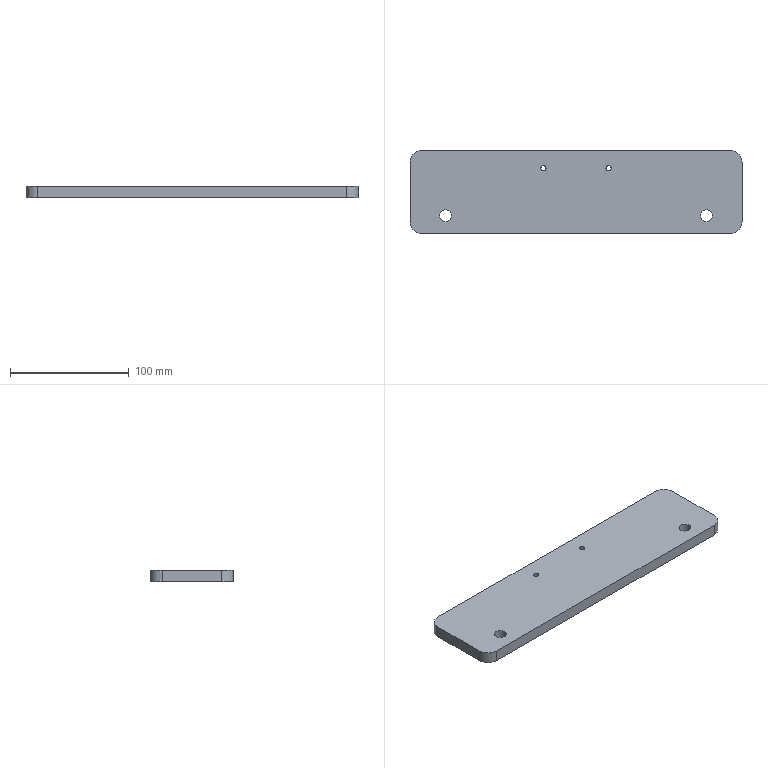Component | SolidWorks | TelescopicCylinderFixedLead-outPlate-1 | 1 solid | 24 faces | box 280 x 70 x 10 mm | volume 192937 mm3 | cylinder 16 | plane 8 | commonest cylinder face diameters 8 x4 4.5 x4 10 x4 20 x4
build123d program:
from build123d import *

# Parameters (mm, degrees)
SKETCH1_W                                         = 280
SKETCH1_H                                         = 70
BOSS_EXTRUDE1_DEPTH                               = 10
SKETCH2_R                                         = 5
CUT_EXTRUDE1_DEPTH                                = 10
FILLET1_R                                         = 10
HOLE_SIZE_ACCORDING_TO_HEXAGON_SOCKET_D           = 4.5
HOLE_SIZE_ACCORDING_TO_HEXAGON_SOCKET_CBORE_D     = 8
HOLE_SIZE_ACCORDING_TO_HEXAGON_SOCKET_CBORE_DEPTH = 4.6


with BuildPart() as part:
    # Sketch1 → Boss-Extrude1 (new body)
    with BuildSketch(Plane.XY):
        with Locations((140, 35)):
            Rectangle(SKETCH1_W, SKETCH1_H)
    extrude(amount=BOSS_EXTRUDE1_DEPTH)

    # Sketch2 → Cut-Extrude1 (cut)
    with BuildSketch(Plane.XY.offset(10)):
        with Locations((30, 55)):
            Circle(SKETCH2_R)
        with Locations((250, 55)):
            Circle(SKETCH2_R)
    extrude(amount=-CUT_EXTRUDE1_DEPTH, mode=Mode.SUBTRACT)

    # Fillet1
    fillet1_edges = [part.edges().sort_by_distance(p)[0] for p in [
        (0, 70, 5),
        (280, 70, 5),
        (280, 0, 5),
        (0, 0, 5),
    ]]
    fillet(fillet1_edges, radius=FILLET1_R)

    # Hole Size _According to_ Hexagon Socket (through all)
    with Locations(Plane(origin=(112.5, 15, 0), x_dir=(-1, 0, 0), z_dir=(0, 0, -1))):
        with Locations((0, 0), (-55, 0)):
            CounterBoreHole(HOLE_SIZE_ACCORDING_TO_HEXAGON_SOCKET_D / 2, HOLE_SIZE_ACCORDING_TO_HEXAGON_SOCKET_CBORE_D / 2, HOLE_SIZE_ACCORDING_TO_HEXAGON_SOCKET_CBORE_DEPTH)


solid = part.part

# Placed as in the assembly
solid = solid.moved(Location((280, -164.228, 0), (0, 0, 180)))
STEP:
#1=COLOUR_RGB('',0.7922,0.8196,0.9333);
#2=FILL_AREA_STYLE_COLOUR('',#1);
#3=FILL_AREA_STYLE('',(#2));
#4=SURFACE_STYLE_FILL_AREA(#3);
#5=SURFACE_SIDE_STYLE('',(#4));
#6=SURFACE_STYLE_USAGE(.BOTH.,#5);
#7=PRESENTATION_STYLE_ASSIGNMENT((#6));
#8=CARTESIAN_POINT('',(6.437,-7.056,0.1811));
#9=VERTEX_POINT('',#8);
#10=CARTESIAN_POINT('',(6.752,-7.056,0.1811));
#11=VERTEX_POINT('',#10);
#12=CARTESIAN_POINT('',(6.594,-7.056,0.1811));
#13=DIRECTION('',(0.,-0.,-1.));
#14=DIRECTION('',(1.,0.,0.));
#15=AXIS2_PLACEMENT_3D('',#12,#13,#14);
#16=CIRCLE('',#15,0.1575);
#17=EDGE_CURVE('',#9,#11,#16,.T.);
#18=ORIENTED_EDGE('',*,*,#17,.F.);
#19=CARTESIAN_POINT('',(6.437,-7.056,0.));
#20=VERTEX_POINT('',#19);
#21=CARTESIAN_POINT('',(6.437,-7.056,0.));
#22=DIRECTION('',(0.,-0.,-1.));
#23=VECTOR('',#22,39.37);
#24=LINE('',#21,#23);
#25=EDGE_CURVE('',#9,#20,#24,.T.);
#26=ORIENTED_EDGE('',*,*,#25,.T.);
#27=CARTESIAN_POINT('',(6.752,-7.056,0.));
#28=VERTEX_POINT('',#27);
#29=CARTESIAN_POINT('',(6.594,-7.056,0.));
#30=DIRECTION('',(0.,-0.,-1.));
#31=DIRECTION('',(1.,0.,0.));
#32=AXIS2_PLACEMENT_3D('',#29,#30,#31);
#33=CIRCLE('',#32,0.1575);
#34=EDGE_CURVE('',#20,#28,#33,.T.);
#35=ORIENTED_EDGE('',*,*,#34,.T.);
#36=CARTESIAN_POINT('',(6.752,-7.056,0.));
#37=DIRECTION('',(0.,-0.,-1.));
#38=VECTOR('',#37,39.37);
#39=LINE('',#36,#38);
#40=EDGE_CURVE('',#11,#28,#39,.T.);
#41=ORIENTED_EDGE('',*,*,#40,.F.);
#42=EDGE_LOOP('',(#18,#26,#35,#41));
#43=FACE_OUTER_BOUND('',#42,.T.);
#44=CARTESIAN_POINT('',(6.594,-7.056,0.));
#45=DIRECTION('',(0.,-0.,-1.));
#46=DIRECTION('',(1.,0.,0.));
#47=AXIS2_PLACEMENT_3D('',#44,#45,#46);
#48=CYLINDRICAL_SURFACE('',#47,0.1575);
#49=ADVANCED_FACE('',(#43),#48,.F.);
#50=CARTESIAN_POINT('',(6.506,-7.056,0.3937));
#51=VERTEX_POINT('',#50);
#52=CARTESIAN_POINT('',(6.683,-7.056,0.3937));
#53=VERTEX_POINT('',#52);
#54=CARTESIAN_POINT('',(6.594,-7.056,0.3937));
#55=DIRECTION('',(0.,-0.,-1.));
#56=DIRECTION('',(1.,0.,0.));
#57=AXIS2_PLACEMENT_3D('',#54,#55,#56);
#58=CIRCLE('',#57,0.08858);
#59=EDGE_CURVE('',#51,#53,#58,.T.);
#60=ORIENTED_EDGE('',*,*,#59,.F.);
#61=CARTESIAN_POINT('',(6.506,-7.056,0.1811));
#62=VERTEX_POINT('',#61);
#63=CARTESIAN_POINT('',(6.506,-7.056,0.));
#64=DIRECTION('',(0.,-0.,-1.));
#65=VECTOR('',#64,39.37);
#66=LINE('',#63,#65);
#67=EDGE_CURVE('',#51,#62,#66,.T.);
#68=ORIENTED_EDGE('',*,*,#67,.T.);
#69=CARTESIAN_POINT('',(6.683,-7.056,0.1811));
#70=VERTEX_POINT('',#69);
#71=CARTESIAN_POINT('',(6.594,-7.056,0.1811));
#72=DIRECTION('',(0.,-0.,-1.));
#73=DIRECTION('',(1.,0.,0.));
#74=AXIS2_PLACEMENT_3D('',#71,#72,#73);
#75=CIRCLE('',#74,0.08858);
#76=EDGE_CURVE('',#62,#70,#75,.T.);
#77=ORIENTED_EDGE('',*,*,#76,.T.);
#78=CARTESIAN_POINT('',(6.683,-7.056,0.));
#79=DIRECTION('',(0.,-0.,-1.));
#80=VECTOR('',#79,39.37);
#81=LINE('',#78,#80);
#82=EDGE_CURVE('',#53,#70,#81,.T.);
#83=ORIENTED_EDGE('',*,*,#82,.F.);
#84=EDGE_LOOP('',(#60,#68,#77,#83));
#85=FACE_OUTER_BOUND('',#84,.T.);
#86=CARTESIAN_POINT('',(6.594,-7.056,0.));
#87=DIRECTION('',(0.,-0.,-1.));
#88=DIRECTION('',(1.,0.,0.));
#89=AXIS2_PLACEMENT_3D('',#86,#87,#88);
#90=CYLINDRICAL_SURFACE('',#89,0.08858);
#91=ADVANCED_FACE('',(#85),#90,.F.);
#92=CARTESIAN_POINT('',(4.272,-7.056,0.1811));
#93=VERTEX_POINT('',#92);
#94=CARTESIAN_POINT('',(4.587,-7.056,0.1811));
#95=VERTEX_POINT('',#94);
#96=CARTESIAN_POINT('',(4.429,-7.056,0.1811));
#97=DIRECTION('',(0.,-0.,-1.));
#98=DIRECTION('',(1.,0.,0.));
#99=AXIS2_PLACEMENT_3D('',#96,#97,#98);
#100=CIRCLE('',#99,0.1575);
#101=EDGE_CURVE('',#93,#95,#100,.T.);
#102=ORIENTED_EDGE('',*,*,#101,.F.);
#103=CARTESIAN_POINT('',(4.272,-7.056,0.));
#104=VERTEX_POINT('',#103);
#105=CARTESIAN_POINT('',(4.272,-7.056,0.));
#106=DIRECTION('',(0.,-0.,-1.));
#107=VECTOR('',#106,39.37);
#108=LINE('',#105,#107);
#109=EDGE_CURVE('',#93,#104,#108,.T.);
#110=ORIENTED_EDGE('',*,*,#109,.T.);
#111=CARTESIAN_POINT('',(4.587,-7.056,0.));
#112=VERTEX_POINT('',#111);
#113=CARTESIAN_POINT('',(4.429,-7.056,0.));
#114=DIRECTION('',(0.,-0.,-1.));
#115=DIRECTION('',(1.,0.,0.));
#116=AXIS2_PLACEMENT_3D('',#113,#114,#115);
#117=CIRCLE('',#116,0.1575);
#118=EDGE_CURVE('',#104,#112,#117,.T.);
#119=ORIENTED_EDGE('',*,*,#118,.T.);
#120=CARTESIAN_POINT('',(4.587,-7.056,0.));
#121=DIRECTION('',(0.,-0.,-1.));
#122=VECTOR('',#121,39.37);
#123=LINE('',#120,#122);
#124=EDGE_CURVE('',#95,#112,#123,.T.);
#125=ORIENTED_EDGE('',*,*,#124,.F.);
#126=EDGE_LOOP('',(#102,#110,#119,#125));
#127=FACE_OUTER_BOUND('',#126,.T.);
#128=CARTESIAN_POINT('',(4.429,-7.056,0.));
#129=DIRECTION('',(0.,-0.,-1.));
#130=DIRECTION('',(1.,0.,0.));
#131=AXIS2_PLACEMENT_3D('',#128,#129,#130);
#132=CYLINDRICAL_SURFACE('',#131,0.1575);
#133=ADVANCED_FACE('',(#127),#132,.F.);
#134=CARTESIAN_POINT('',(4.341,-7.056,0.3937));
#135=VERTEX_POINT('',#134);
#136=CARTESIAN_POINT('',(4.518,-7.056,0.3937));
#137=VERTEX_POINT('',#136);
#138=CARTESIAN_POINT('',(4.429,-7.056,0.3937));
#139=DIRECTION('',(0.,-0.,-1.));
#140=DIRECTION('',(1.,0.,0.));
#141=AXIS2_PLACEMENT_3D('',#138,#139,#140);
#142=CIRCLE('',#141,0.08858);
#143=EDGE_CURVE('',#135,#137,#142,.T.);
#144=ORIENTED_EDGE('',*,*,#143,.F.);
#145=CARTESIAN_POINT('',(4.341,-7.056,0.1811));
#146=VERTEX_POINT('',#145);
#147=CARTESIAN_POINT('',(4.341,-7.056,0.));
#148=DIRECTION('',(0.,-0.,-1.));
#149=VECTOR('',#148,39.37);
#150=LINE('',#147,#149);
#151=EDGE_CURVE('',#135,#146,#150,.T.);
#152=ORIENTED_EDGE('',*,*,#151,.T.);
#153=CARTESIAN_POINT('',(4.518,-7.056,0.1811));
#154=VERTEX_POINT('',#153);
#155=CARTESIAN_POINT('',(4.429,-7.056,0.1811));
#156=DIRECTION('',(0.,-0.,-1.));
#157=DIRECTION('',(1.,0.,0.));
#158=AXIS2_PLACEMENT_3D('',#155,#156,#157);
#159=CIRCLE('',#158,0.08858);
#160=EDGE_CURVE('',#146,#154,#159,.T.);
#161=ORIENTED_EDGE('',*,*,#160,.T.);
#162=CARTESIAN_POINT('',(4.518,-7.056,0.));
#163=DIRECTION('',(0.,-0.,-1.));
#164=VECTOR('',#163,39.37);
#165=LINE('',#162,#164);
#166=EDGE_CURVE('',#137,#154,#165,.T.);
#167=ORIENTED_EDGE('',*,*,#166,.F.);
#168=EDGE_LOOP('',(#144,#152,#161,#167));
#169=FACE_OUTER_BOUND('',#168,.T.);
#170=CARTESIAN_POINT('',(4.429,-7.056,0.));
#171=DIRECTION('',(0.,-0.,-1.));
#172=DIRECTION('',(1.,0.,0.));
#173=AXIS2_PLACEMENT_3D('',#170,#171,#172);
#174=CYLINDRICAL_SURFACE('',#173,0.08858);
#175=ADVANCED_FACE('',(#169),#174,.F.);
#176=CARTESIAN_POINT('',(1.378,-8.631,0.));
#177=VERTEX_POINT('',#176);
#178=CARTESIAN_POINT('',(0.9843,-8.631,0.));
#179=VERTEX_POINT('',#178);
#180=CARTESIAN_POINT('',(1.181,-8.631,0.));
#181=DIRECTION('',(-0.,0.,1.));
#182=DIRECTION('',(-1.,0.,-0.));
#183=AXIS2_PLACEMENT_3D('',#180,#181,#182);
#184=CIRCLE('',#183,0.1969);
#185=EDGE_CURVE('',#177,#179,#184,.T.);
#186=ORIENTED_EDGE('',*,*,#185,.F.);
#187=CARTESIAN_POINT('',(1.378,-8.631,0.3937));
#188=VERTEX_POINT('',#187);
#189=CARTESIAN_POINT('',(1.378,-8.631,0.));
#190=DIRECTION('',(-0.,0.,1.));
#191=VECTOR('',#190,39.37);
#192=LINE('',#189,#191);
#193=EDGE_CURVE('',#177,#188,#192,.T.);
#194=ORIENTED_EDGE('',*,*,#193,.T.);
#195=CARTESIAN_POINT('',(0.9843,-8.631,0.3937));
#196=VERTEX_POINT('',#195);
#197=CARTESIAN_POINT('',(1.181,-8.631,0.3937));
#198=DIRECTION('',(-0.,0.,1.));
#199=DIRECTION('',(-1.,0.,0.));
#200=AXIS2_PLACEMENT_3D('',#197,#198,#199);
#201=CIRCLE('',#200,0.1969);
#202=EDGE_CURVE('',#188,#196,#201,.T.);
#203=ORIENTED_EDGE('',*,*,#202,.T.);
#204=CARTESIAN_POINT('',(0.9843,-8.631,0.));
#205=DIRECTION('',(-0.,0.,1.));
#206=VECTOR('',#205,39.37);
#207=LINE('',#204,#206);
#208=EDGE_CURVE('',#179,#196,#207,.T.);
#209=ORIENTED_EDGE('',*,*,#208,.F.);
#210=EDGE_LOOP('',(#186,#194,#203,#209));
#211=FACE_OUTER_BOUND('',#210,.T.);
#212=CARTESIAN_POINT('',(1.181,-8.631,0.));
#213=DIRECTION('',(-0.,0.,1.));
#214=DIRECTION('',(-1.,0.,-0.));
#215=AXIS2_PLACEMENT_3D('',#212,#213,#214);
#216=CYLINDRICAL_SURFACE('',#215,0.1969);
#217=ADVANCED_FACE('',(#211),#216,.F.);
#218=CARTESIAN_POINT('',(10.039,-8.631,0.));
#219=VERTEX_POINT('',#218);
#220=CARTESIAN_POINT('',(9.646,-8.631,0.));
#221=VERTEX_POINT('',#220);
#222=CARTESIAN_POINT('',(9.843,-8.631,0.));
#223=DIRECTION('',(-0.,0.,1.));
#224=DIRECTION('',(-1.,0.,-0.));
#225=AXIS2_PLACEMENT_3D('',#222,#223,#224);
#226=CIRCLE('',#225,0.1969);
#227=EDGE_CURVE('',#219,#221,#226,.T.);
#228=ORIENTED_EDGE('',*,*,#227,.F.);
#229=CARTESIAN_POINT('',(10.039,-8.631,0.3937));
#230=VERTEX_POINT('',#229);
#231=CARTESIAN_POINT('',(10.039,-8.631,0.));
#232=DIRECTION('',(-0.,0.,1.));
#233=VECTOR('',#232,39.37);
#234=LINE('',#231,#233);
#235=EDGE_CURVE('',#219,#230,#234,.T.);
#236=ORIENTED_EDGE('',*,*,#235,.T.);
#237=CARTESIAN_POINT('',(9.646,-8.631,0.3937));
#238=VERTEX_POINT('',#237);
#239=CARTESIAN_POINT('',(9.843,-8.631,0.3937));
#240=DIRECTION('',(-0.,0.,1.));
#241=DIRECTION('',(-1.,0.,0.));
#242=AXIS2_PLACEMENT_3D('',#239,#240,#241);
#243=CIRCLE('',#242,0.1969);
#244=EDGE_CURVE('',#230,#238,#243,.T.);
#245=ORIENTED_EDGE('',*,*,#244,.T.);
#246=CARTESIAN_POINT('',(9.646,-8.631,0.));
#247=DIRECTION('',(-0.,0.,1.));
#248=VECTOR('',#247,39.37);
#249=LINE('',#246,#248);
#250=EDGE_CURVE('',#221,#238,#249,.T.);
#251=ORIENTED_EDGE('',*,*,#250,.F.);
#252=EDGE_LOOP('',(#228,#236,#245,#251));
#253=FACE_OUTER_BOUND('',#252,.T.);
#254=CARTESIAN_POINT('',(9.843,-8.631,0.));
#255=DIRECTION('',(-0.,0.,1.));
#256=DIRECTION('',(-1.,0.,-0.));
#257=AXIS2_PLACEMENT_3D('',#254,#255,#256);
#258=CYLINDRICAL_SURFACE('',#257,0.1969);
#259=ADVANCED_FACE('',(#253),#258,.F.);
#260=CARTESIAN_POINT('',(11.024,-8.828,0.));
#261=VERTEX_POINT('',#260);
#262=CARTESIAN_POINT('',(11.024,-6.859,0.));
#263=VERTEX_POINT('',#262);
#264=CARTESIAN_POINT('',(11.024,-6.466,0.));
#265=DIRECTION('',(-0.,1.,-0.));
#266=VECTOR('',#265,39.37);
#267=LINE('',#264,#266);
#268=EDGE_CURVE('',#261,#263,#267,.T.);
#269=ORIENTED_EDGE('',*,*,#268,.T.);
#270=CARTESIAN_POINT('',(11.024,-6.859,0.3937));
#271=VERTEX_POINT('',#270);
#272=CARTESIAN_POINT('',(11.024,-6.859,0.3937));
#273=DIRECTION('',(-0.,0.,1.));
#274=VECTOR('',#273,39.37);
#275=LINE('',#272,#274);
#276=EDGE_CURVE('',#263,#271,#275,.T.);
#277=ORIENTED_EDGE('',*,*,#276,.T.);
#278=CARTESIAN_POINT('',(11.024,-8.828,0.3937));
#279=VERTEX_POINT('',#278);
#280=CARTESIAN_POINT('',(11.024,-6.466,0.3937));
#281=DIRECTION('',(-0.,1.,-0.));
#282=VECTOR('',#281,39.37);
#283=LINE('',#280,#282);
#284=EDGE_CURVE('',#279,#271,#283,.T.);
#285=ORIENTED_EDGE('',*,*,#284,.F.);
#286=CARTESIAN_POINT('',(11.024,-8.828,0.3937));
#287=DIRECTION('',(0.,-0.,-1.));
#288=VECTOR('',#287,39.37);
#289=LINE('',#286,#288);
#290=EDGE_CURVE('',#279,#261,#289,.T.);
#291=ORIENTED_EDGE('',*,*,#290,.T.);
#292=EDGE_LOOP('',(#269,#277,#285,#291));
#293=FACE_OUTER_BOUND('',#292,.T.);
#294=CARTESIAN_POINT('',(11.024,-6.466,0.3937));
#295=DIRECTION('',(-1.,-0.,-0.));
#296=DIRECTION('',(0.,-0.,-1.));
#297=AXIS2_PLACEMENT_3D('',#294,#295,#296);
#298=PLANE('',#297);
#299=ADVANCED_FACE('',(#293),#298,.F.);
#300=CARTESIAN_POINT('',(10.63,-6.466,0.));
#301=VERTEX_POINT('',#300);
#302=CARTESIAN_POINT('',(0.3937,-6.466,0.));
#303=VERTEX_POINT('',#302);
#304=CARTESIAN_POINT('',(11.024,-6.466,0.));
#305=DIRECTION('',(-1.,-0.,-0.));
#306=VECTOR('',#305,39.37);
#307=LINE('',#304,#306);
#308=EDGE_CURVE('',#301,#303,#307,.T.);
#309=ORIENTED_EDGE('',*,*,#308,.T.);
#310=CARTESIAN_POINT('',(0.3937,-6.466,0.3937));
#311=VERTEX_POINT('',#310);
#312=CARTESIAN_POINT('',(0.3937,-6.466,0.3937));
#313=DIRECTION('',(-0.,0.,1.));
#314=VECTOR('',#313,39.37);
#315=LINE('',#312,#314);
#316=EDGE_CURVE('',#303,#311,#315,.T.);
#317=ORIENTED_EDGE('',*,*,#316,.T.);
#318=CARTESIAN_POINT('',(10.63,-6.466,0.3937));
#319=VERTEX_POINT('',#318);
#320=CARTESIAN_POINT('',(11.024,-6.466,0.3937));
#321=DIRECTION('',(-1.,-0.,-0.));
#322=VECTOR('',#321,39.37);
#323=LINE('',#320,#322);
#324=EDGE_CURVE('',#319,#311,#323,.T.);
#325=ORIENTED_EDGE('',*,*,#324,.F.);
#326=CARTESIAN_POINT('',(10.63,-6.466,0.3937));
#327=DIRECTION('',(0.,-0.,-1.));
#328=VECTOR('',#327,39.37);
#329=LINE('',#326,#328);
#330=EDGE_CURVE('',#319,#301,#329,.T.);
#331=ORIENTED_EDGE('',*,*,#330,.T.);
#332=EDGE_LOOP('',(#309,#317,#325,#331));
#333=FACE_OUTER_BOUND('',#332,.T.);
#334=CARTESIAN_POINT('',(11.024,-6.466,0.3937));
#335=DIRECTION('',(0.,-1.,0.));
#336=DIRECTION('',(-0.,0.,1.));
#337=AXIS2_PLACEMENT_3D('',#334,#335,#336);
#338=PLANE('',#337);
#339=ADVANCED_FACE('',(#333),#338,.F.);
#340=CARTESIAN_POINT('',(0.,-6.859,0.));
#341=VERTEX_POINT('',#340);
#342=CARTESIAN_POINT('',(0.,-8.828,0.));
#343=VERTEX_POINT('',#342);
#344=CARTESIAN_POINT('',(0.,-6.466,0.));
#345=DIRECTION('',(0.,-1.,0.));
#346=VECTOR('',#345,39.37);
#347=LINE('',#344,#346);
#348=EDGE_CURVE('',#341,#343,#347,.T.);
#349=ORIENTED_EDGE('',*,*,#348,.T.);
#350=CARTESIAN_POINT('',(0.,-8.828,0.3937));
#351=VERTEX_POINT('',#350);
#352=CARTESIAN_POINT('',(0.,-8.828,0.3937));
#353=DIRECTION('',(-0.,0.,1.));
#354=VECTOR('',#353,39.37);
#355=LINE('',#352,#354);
#356=EDGE_CURVE('',#343,#351,#355,.T.);
#357=ORIENTED_EDGE('',*,*,#356,.T.);
#358=CARTESIAN_POINT('',(0.,-6.859,0.3937));
#359=VERTEX_POINT('',#358);
#360=CARTESIAN_POINT('',(0.,-6.466,0.3937));
#361=DIRECTION('',(0.,-1.,0.));
#362=VECTOR('',#361,39.37);
#363=LINE('',#360,#362);
#364=EDGE_CURVE('',#359,#351,#363,.T.);
#365=ORIENTED_EDGE('',*,*,#364,.F.);
#366=CARTESIAN_POINT('',(0.,-6.859,0.3937));
#367=DIRECTION('',(0.,-0.,-1.));
#368=VECTOR('',#367,39.37);
#369=LINE('',#366,#368);
#370=EDGE_CURVE('',#359,#341,#369,.T.);
#371=ORIENTED_EDGE('',*,*,#370,.T.);
#372=EDGE_LOOP('',(#349,#357,#365,#371));
#373=FACE_OUTER_BOUND('',#372,.T.);
#374=CARTESIAN_POINT('',(0.,-6.466,0.3937));
#375=DIRECTION('',(1.,0.,0.));
#376=DIRECTION('',(-0.,0.,1.));
#377=AXIS2_PLACEMENT_3D('',#374,#375,#376);
#378=PLANE('',#377);
#379=ADVANCED_FACE('',(#373),#378,.F.);
#380=CARTESIAN_POINT('',(0.3937,-9.222,0.3937));
#381=VERTEX_POINT('',#380);
#382=CARTESIAN_POINT('',(10.63,-9.222,0.3937));
#383=VERTEX_POINT('',#382);
#384=CARTESIAN_POINT('',(11.024,-9.222,0.3937));
#385=DIRECTION('',(1.,0.,0.));
#386=VECTOR('',#385,39.37);
#387=LINE('',#384,#386);
#388=EDGE_CURVE('',#381,#383,#387,.T.);
#389=ORIENTED_EDGE('',*,*,#388,.F.);
#390=CARTESIAN_POINT('',(0.3937,-9.222,0.));
#391=VERTEX_POINT('',#390);
#392=CARTESIAN_POINT('',(0.3937,-9.222,0.3937));
#393=DIRECTION('',(0.,-0.,-1.));
#394=VECTOR('',#393,39.37);
#395=LINE('',#392,#394);
#396=EDGE_CURVE('',#381,#391,#395,.T.);
#397=ORIENTED_EDGE('',*,*,#396,.T.);
#398=CARTESIAN_POINT('',(10.63,-9.222,0.));
#399=VERTEX_POINT('',#398);
#400=CARTESIAN_POINT('',(11.024,-9.222,0.));
#401=DIRECTION('',(1.,0.,0.));
#402=VECTOR('',#401,39.37);
#403=LINE('',#400,#402);
#404=EDGE_CURVE('',#391,#399,#403,.T.);
#405=ORIENTED_EDGE('',*,*,#404,.T.);
#406=CARTESIAN_POINT('',(10.63,-9.222,0.3937));
#407=DIRECTION('',(-0.,0.,1.));
#408=VECTOR('',#407,39.37);
#409=LINE('',#406,#408);
#410=EDGE_CURVE('',#399,#383,#409,.T.);
#411=ORIENTED_EDGE('',*,*,#410,.T.);
#412=EDGE_LOOP('',(#389,#397,#405,#411));
#413=FACE_OUTER_BOUND('',#412,.T.);
#414=CARTESIAN_POINT('',(11.024,-9.222,0.3937));
#415=DIRECTION('',(-0.,1.,-0.));
#416=DIRECTION('',(0.,-0.,-1.));
#417=AXIS2_PLACEMENT_3D('',#414,#415,#416);
#418=PLANE('',#417);
#419=ADVANCED_FACE('',(#413),#418,.F.);
#420=CARTESIAN_POINT('',(6.594,-7.056,0.3937));
#421=DIRECTION('',(0.,-0.,-1.));
#422=DIRECTION('',(1.,0.,0.));
#423=AXIS2_PLACEMENT_3D('',#420,#421,#422);
#424=CIRCLE('',#423,0.08858);
#425=EDGE_CURVE('',#53,#51,#424,.T.);
#426=ORIENTED_EDGE('',*,*,#425,.T.);
#427=ORIENTED_EDGE('',*,*,#59,.T.);
#428=EDGE_LOOP('',(#426,#427));
#429=FACE_BOUND('',#428,.T.);
#430=CARTESIAN_POINT('',(4.429,-7.056,0.3937));
#431=DIRECTION('',(0.,-0.,-1.));
#432=DIRECTION('',(1.,0.,0.));
#433=AXIS2_PLACEMENT_3D('',#430,#431,#432);
#434=CIRCLE('',#433,0.08858);
#435=EDGE_CURVE('',#137,#135,#434,.T.);
#436=ORIENTED_EDGE('',*,*,#435,.T.);
#437=ORIENTED_EDGE('',*,*,#143,.T.);
#438=EDGE_LOOP('',(#436,#437));
#439=FACE_BOUND('',#438,.T.);
#440=CARTESIAN_POINT('',(1.181,-8.631,0.3937));
#441=DIRECTION('',(-0.,0.,1.));
#442=DIRECTION('',(-1.,0.,0.));
#443=AXIS2_PLACEMENT_3D('',#440,#441,#442);
#444=CIRCLE('',#443,0.1969);
#445=EDGE_CURVE('',#196,#188,#444,.T.);
#446=ORIENTED_EDGE('',*,*,#445,.F.);
#447=ORIENTED_EDGE('',*,*,#202,.F.);
#448=EDGE_LOOP('',(#446,#447));
#449=FACE_BOUND('',#448,.T.);
#450=CARTESIAN_POINT('',(9.843,-8.631,0.3937));
#451=DIRECTION('',(-0.,0.,1.));
#452=DIRECTION('',(-1.,0.,0.));
#453=AXIS2_PLACEMENT_3D('',#450,#451,#452);
#454=CIRCLE('',#453,0.1969);
#455=EDGE_CURVE('',#238,#230,#454,.T.);
#456=ORIENTED_EDGE('',*,*,#455,.F.);
#457=ORIENTED_EDGE('',*,*,#244,.F.);
#458=EDGE_LOOP('',(#456,#457));
#459=FACE_BOUND('',#458,.T.);
#460=ORIENTED_EDGE('',*,*,#364,.T.);
#461=CARTESIAN_POINT('',(0.3937,-8.828,0.3937));
#462=DIRECTION('',(-0.,0.,1.));
#463=DIRECTION('',(1.,0.,0.));
#464=AXIS2_PLACEMENT_3D('',#461,#462,#463);
#465=CIRCLE('',#464,0.3937);
#466=EDGE_CURVE('',#351,#381,#465,.T.);
#467=ORIENTED_EDGE('',*,*,#466,.T.);
#468=ORIENTED_EDGE('',*,*,#388,.T.);
#469=CARTESIAN_POINT('',(10.63,-8.828,0.3937));
#470=DIRECTION('',(-0.,0.,1.));
#471=DIRECTION('',(1.,0.,0.));
#472=AXIS2_PLACEMENT_3D('',#469,#470,#471);
#473=CIRCLE('',#472,0.3937);
#474=EDGE_CURVE('',#383,#279,#473,.T.);
#475=ORIENTED_EDGE('',*,*,#474,.T.);
#476=ORIENTED_EDGE('',*,*,#284,.T.);
#477=CARTESIAN_POINT('',(10.63,-6.859,0.3937));
#478=DIRECTION('',(-0.,0.,1.));
#479=DIRECTION('',(1.,0.,0.));
#480=AXIS2_PLACEMENT_3D('',#477,#478,#479);
#481=CIRCLE('',#480,0.3937);
#482=EDGE_CURVE('',#271,#319,#481,.T.);
#483=ORIENTED_EDGE('',*,*,#482,.T.);
#484=ORIENTED_EDGE('',*,*,#324,.T.);
#485=CARTESIAN_POINT('',(0.3937,-6.859,0.3937));
#486=DIRECTION('',(-0.,0.,1.));
#487=DIRECTION('',(1.,0.,0.));
#488=AXIS2_PLACEMENT_3D('',#485,#486,#487);
#489=CIRCLE('',#488,0.3937);
#490=EDGE_CURVE('',#311,#359,#489,.T.);
#491=ORIENTED_EDGE('',*,*,#490,.T.);
#492=EDGE_LOOP('',(#460,#467,#468,#475,#476,#483,#484,#491));
#493=FACE_OUTER_BOUND('',#492,.T.);
#494=CARTESIAN_POINT('',(11.024,-6.466,0.3937));
#495=DIRECTION('',(0.,-0.,-1.));
#496=DIRECTION('',(1.,0.,0.));
#497=AXIS2_PLACEMENT_3D('',#494,#495,#496);
#498=PLANE('',#497);
#499=ADVANCED_FACE('',(#429,#439,#449,#459,#493),#498,.F.);
#500=CARTESIAN_POINT('',(6.594,-7.056,0.));
#501=DIRECTION('',(0.,-0.,-1.));
#502=DIRECTION('',(1.,0.,0.));
#503=AXIS2_PLACEMENT_3D('',#500,#501,#502);
#504=CIRCLE('',#503,0.1575);
#505=EDGE_CURVE('',#28,#20,#504,.T.);
#506=ORIENTED_EDGE('',*,*,#505,.F.);
#507=ORIENTED_EDGE('',*,*,#34,.F.);
#508=EDGE_LOOP('',(#506,#507));
#509=FACE_BOUND('',#508,.T.);
#510=CARTESIAN_POINT('',(4.429,-7.056,0.));
#511=DIRECTION('',(0.,-0.,-1.));
#512=DIRECTION('',(1.,0.,0.));
#513=AXIS2_PLACEMENT_3D('',#510,#511,#512);
#514=CIRCLE('',#513,0.1575);
#515=EDGE_CURVE('',#112,#104,#514,.T.);
#516=ORIENTED_EDGE('',*,*,#515,.F.);
#517=ORIENTED_EDGE('',*,*,#118,.F.);
#518=EDGE_LOOP('',(#516,#517));
#519=FACE_BOUND('',#518,.T.);
#520=CARTESIAN_POINT('',(1.181,-8.631,0.));
#521=DIRECTION('',(-0.,0.,1.));
#522=DIRECTION('',(-1.,0.,-0.));
#523=AXIS2_PLACEMENT_3D('',#520,#521,#522);
#524=CIRCLE('',#523,0.1969);
#525=EDGE_CURVE('',#179,#177,#524,.T.);
#526=ORIENTED_EDGE('',*,*,#525,.T.);
#527=ORIENTED_EDGE('',*,*,#185,.T.);
#528=EDGE_LOOP('',(#526,#527));
#529=FACE_BOUND('',#528,.T.);
#530=CARTESIAN_POINT('',(9.843,-8.631,0.));
#531=DIRECTION('',(-0.,0.,1.));
#532=DIRECTION('',(-1.,0.,-0.));
#533=AXIS2_PLACEMENT_3D('',#530,#531,#532);
#534=CIRCLE('',#533,0.1969);
#535=EDGE_CURVE('',#221,#219,#534,.T.);
#536=ORIENTED_EDGE('',*,*,#535,.T.);
#537=ORIENTED_EDGE('',*,*,#227,.T.);
#538=EDGE_LOOP('',(#536,#537));
#539=FACE_BOUND('',#538,.T.);
#540=ORIENTED_EDGE('',*,*,#404,.F.);
#541=CARTESIAN_POINT('',(0.3937,-8.828,0.));
#542=DIRECTION('',(0.,-0.,-1.));
#543=DIRECTION('',(1.,0.,0.));
#544=AXIS2_PLACEMENT_3D('',#541,#542,#543);
#545=CIRCLE('',#544,0.3937);
#546=EDGE_CURVE('',#391,#343,#545,.T.);
#547=ORIENTED_EDGE('',*,*,#546,.T.);
#548=ORIENTED_EDGE('',*,*,#348,.F.);
#549=CARTESIAN_POINT('',(0.3937,-6.859,0.));
#550=DIRECTION('',(0.,-0.,-1.));
#551=DIRECTION('',(1.,0.,0.));
#552=AXIS2_PLACEMENT_3D('',#549,#550,#551);
#553=CIRCLE('',#552,0.3937);
#554=EDGE_CURVE('',#341,#303,#553,.T.);
#555=ORIENTED_EDGE('',*,*,#554,.T.);
#556=ORIENTED_EDGE('',*,*,#308,.F.);
#557=CARTESIAN_POINT('',(10.63,-6.859,0.));
#558=DIRECTION('',(0.,-0.,-1.));
#559=DIRECTION('',(1.,0.,0.));
#560=AXIS2_PLACEMENT_3D('',#557,#558,#559);
#561=CIRCLE('',#560,0.3937);
#562=EDGE_CURVE('',#301,#263,#561,.T.);
#563=ORIENTED_EDGE('',*,*,#562,.T.);
#564=ORIENTED_EDGE('',*,*,#268,.F.);
#565=CARTESIAN_POINT('',(10.63,-8.828,0.));
#566=DIRECTION('',(0.,-0.,-1.));
#567=DIRECTION('',(1.,0.,0.));
#568=AXIS2_PLACEMENT_3D('',#565,#566,#567);
#569=CIRCLE('',#568,0.3937);
#570=EDGE_CURVE('',#261,#399,#569,.T.);
#571=ORIENTED_EDGE('',*,*,#570,.T.);
#572=EDGE_LOOP('',(#540,#547,#548,#555,#556,#563,#564,#571));
#573=FACE_OUTER_BOUND('',#572,.T.);
#574=CARTESIAN_POINT('',(11.024,-6.466,0.));
#575=DIRECTION('',(0.,-0.,-1.));
#576=DIRECTION('',(1.,0.,0.));
#577=AXIS2_PLACEMENT_3D('',#574,#575,#576);
#578=PLANE('',#577);
#579=ADVANCED_FACE('',(#509,#519,#529,#539,#573),#578,.T.);
#580=ORIENTED_EDGE('',*,*,#235,.F.);
#581=ORIENTED_EDGE('',*,*,#535,.F.);
#582=ORIENTED_EDGE('',*,*,#250,.T.);
#583=ORIENTED_EDGE('',*,*,#455,.T.);
#584=EDGE_LOOP('',(#580,#581,#582,#583));
#585=FACE_OUTER_BOUND('',#584,.T.);
#586=CARTESIAN_POINT('',(9.843,-8.631,0.));
#587=DIRECTION('',(-0.,0.,1.));
#588=DIRECTION('',(-1.,0.,-0.));
#589=AXIS2_PLACEMENT_3D('',#586,#587,#588);
#590=CYLINDRICAL_SURFACE('',#589,0.1969);
#591=ADVANCED_FACE('',(#585),#590,.F.);
#592=ORIENTED_EDGE('',*,*,#193,.F.);
#593=ORIENTED_EDGE('',*,*,#525,.F.);
#594=ORIENTED_EDGE('',*,*,#208,.T.);
#595=ORIENTED_EDGE('',*,*,#445,.T.);
#596=EDGE_LOOP('',(#592,#593,#594,#595));
#597=FACE_OUTER_BOUND('',#596,.T.);
#598=CARTESIAN_POINT('',(1.181,-8.631,0.));
#599=DIRECTION('',(-0.,0.,1.));
#600=DIRECTION('',(-1.,0.,-0.));
#601=AXIS2_PLACEMENT_3D('',#598,#599,#600);
#602=CYLINDRICAL_SURFACE('',#601,0.1969);
#603=ADVANCED_FACE('',(#597),#602,.F.);
#604=ORIENTED_EDGE('',*,*,#466,.F.);
#605=ORIENTED_EDGE('',*,*,#356,.F.);
#606=ORIENTED_EDGE('',*,*,#546,.F.);
#607=ORIENTED_EDGE('',*,*,#396,.F.);
#608=EDGE_LOOP('',(#604,#605,#606,#607));
#609=FACE_OUTER_BOUND('',#608,.T.);
#610=CARTESIAN_POINT('',(0.3937,-8.828,0.3937));
#611=DIRECTION('',(0.,-0.,-1.));
#612=DIRECTION('',(1.,0.,0.));
#613=AXIS2_PLACEMENT_3D('',#610,#611,#612);
#614=CYLINDRICAL_SURFACE('',#613,0.3937);
#615=ADVANCED_FACE('',(#609),#614,.T.);
#616=ORIENTED_EDGE('',*,*,#490,.F.);
#617=ORIENTED_EDGE('',*,*,#316,.F.);
#618=ORIENTED_EDGE('',*,*,#554,.F.);
#619=ORIENTED_EDGE('',*,*,#370,.F.);
#620=EDGE_LOOP('',(#616,#617,#618,#619));
#621=FACE_OUTER_BOUND('',#620,.T.);
#622=CARTESIAN_POINT('',(0.3937,-6.859,0.3937));
#623=DIRECTION('',(0.,-0.,-1.));
#624=DIRECTION('',(1.,0.,0.));
#625=AXIS2_PLACEMENT_3D('',#622,#623,#624);
#626=CYLINDRICAL_SURFACE('',#625,0.3937);
#627=ADVANCED_FACE('',(#621),#626,.T.);
#628=ORIENTED_EDGE('',*,*,#482,.F.);
#629=ORIENTED_EDGE('',*,*,#276,.F.);
#630=ORIENTED_EDGE('',*,*,#562,.F.);
#631=ORIENTED_EDGE('',*,*,#330,.F.);
#632=EDGE_LOOP('',(#628,#629,#630,#631));
#633=FACE_OUTER_BOUND('',#632,.T.);
#634=CARTESIAN_POINT('',(10.63,-6.859,0.3937));
#635=DIRECTION('',(0.,-0.,-1.));
#636=DIRECTION('',(1.,0.,0.));
#637=AXIS2_PLACEMENT_3D('',#634,#635,#636);
#638=CYLINDRICAL_SURFACE('',#637,0.3937);
#639=ADVANCED_FACE('',(#633),#638,.T.);
#640=ORIENTED_EDGE('',*,*,#474,.F.);
#641=ORIENTED_EDGE('',*,*,#410,.F.);
#642=ORIENTED_EDGE('',*,*,#570,.F.);
#643=ORIENTED_EDGE('',*,*,#290,.F.);
#644=EDGE_LOOP('',(#640,#641,#642,#643));
#645=FACE_OUTER_BOUND('',#644,.T.);
#646=CARTESIAN_POINT('',(10.63,-8.828,0.3937));
#647=DIRECTION('',(0.,-0.,-1.));
#648=DIRECTION('',(1.,0.,0.));
#649=AXIS2_PLACEMENT_3D('',#646,#647,#648);
#650=CYLINDRICAL_SURFACE('',#649,0.3937);
#651=ADVANCED_FACE('',(#645),#650,.T.);
#652=ORIENTED_EDGE('',*,*,#151,.F.);
#653=ORIENTED_EDGE('',*,*,#435,.F.);
#654=ORIENTED_EDGE('',*,*,#166,.T.);
#655=CARTESIAN_POINT('',(4.429,-7.056,0.1811));
#656=DIRECTION('',(0.,-0.,-1.));
#657=DIRECTION('',(1.,0.,0.));
#658=AXIS2_PLACEMENT_3D('',#655,#656,#657);
#659=CIRCLE('',#658,0.08858);
#660=EDGE_CURVE('',#154,#146,#659,.T.);
#661=ORIENTED_EDGE('',*,*,#660,.T.);
#662=EDGE_LOOP('',(#652,#653,#654,#661));
#663=FACE_OUTER_BOUND('',#662,.T.);
#664=CARTESIAN_POINT('',(4.429,-7.056,0.));
#665=DIRECTION('',(0.,-0.,-1.));
#666=DIRECTION('',(1.,0.,0.));
#667=AXIS2_PLACEMENT_3D('',#664,#665,#666);
#668=CYLINDRICAL_SURFACE('',#667,0.08858);
#669=ADVANCED_FACE('',(#663),#668,.F.);
#670=ORIENTED_EDGE('',*,*,#660,.F.);
#671=ORIENTED_EDGE('',*,*,#160,.F.);
#672=EDGE_LOOP('',(#670,#671));
#673=FACE_BOUND('',#672,.T.);
#674=CARTESIAN_POINT('',(4.429,-7.056,0.1811));
#675=DIRECTION('',(0.,-0.,-1.));
#676=DIRECTION('',(1.,0.,0.));
#677=AXIS2_PLACEMENT_3D('',#674,#675,#676);
#678=CIRCLE('',#677,0.1575);
#679=EDGE_CURVE('',#95,#93,#678,.T.);
#680=ORIENTED_EDGE('',*,*,#679,.T.);
#681=ORIENTED_EDGE('',*,*,#101,.T.);
#682=EDGE_LOOP('',(#680,#681));
#683=FACE_OUTER_BOUND('',#682,.T.);
#684=CARTESIAN_POINT('',(4.341,-7.056,0.1811));
#685=DIRECTION('',(-0.,0.,1.));
#686=DIRECTION('',(-1.,-0.,-0.));
#687=AXIS2_PLACEMENT_3D('',#684,#685,#686);
#688=PLANE('',#687);
#689=ADVANCED_FACE('',(#673,#683),#688,.F.);
#690=ORIENTED_EDGE('',*,*,#109,.F.);
#691=ORIENTED_EDGE('',*,*,#679,.F.);
#692=ORIENTED_EDGE('',*,*,#124,.T.);
#693=ORIENTED_EDGE('',*,*,#515,.T.);
#694=EDGE_LOOP('',(#690,#691,#692,#693));
#695=FACE_OUTER_BOUND('',#694,.T.);
#696=CARTESIAN_POINT('',(4.429,-7.056,0.));
#697=DIRECTION('',(0.,-0.,-1.));
#698=DIRECTION('',(1.,0.,0.));
#699=AXIS2_PLACEMENT_3D('',#696,#697,#698);
#700=CYLINDRICAL_SURFACE('',#699,0.1575);
#701=ADVANCED_FACE('',(#695),#700,.F.);
#702=ORIENTED_EDGE('',*,*,#67,.F.);
#703=ORIENTED_EDGE('',*,*,#425,.F.);
#704=ORIENTED_EDGE('',*,*,#82,.T.);
#705=CARTESIAN_POINT('',(6.594,-7.056,0.1811));
#706=DIRECTION('',(0.,-0.,-1.));
#707=DIRECTION('',(1.,0.,0.));
#708=AXIS2_PLACEMENT_3D('',#705,#706,#707);
#709=CIRCLE('',#708,0.08858);
#710=EDGE_CURVE('',#70,#62,#709,.T.);
#711=ORIENTED_EDGE('',*,*,#710,.T.);
#712=EDGE_LOOP('',(#702,#703,#704,#711));
#713=FACE_OUTER_BOUND('',#712,.T.);
#714=CARTESIAN_POINT('',(6.594,-7.056,0.));
#715=DIRECTION('',(0.,-0.,-1.));
#716=DIRECTION('',(1.,0.,0.));
#717=AXIS2_PLACEMENT_3D('',#714,#715,#716);
#718=CYLINDRICAL_SURFACE('',#717,0.08858);
#719=ADVANCED_FACE('',(#713),#718,.F.);
#720=ORIENTED_EDGE('',*,*,#710,.F.);
#721=ORIENTED_EDGE('',*,*,#76,.F.);
#722=EDGE_LOOP('',(#720,#721));
#723=FACE_BOUND('',#722,.T.);
#724=CARTESIAN_POINT('',(6.594,-7.056,0.1811));
#725=DIRECTION('',(0.,-0.,-1.));
#726=DIRECTION('',(1.,0.,0.));
#727=AXIS2_PLACEMENT_3D('',#724,#725,#726);
#728=CIRCLE('',#727,0.1575);
#729=EDGE_CURVE('',#11,#9,#728,.T.);
#730=ORIENTED_EDGE('',*,*,#729,.T.);
#731=ORIENTED_EDGE('',*,*,#17,.T.);
#732=EDGE_LOOP('',(#730,#731));
#733=FACE_OUTER_BOUND('',#732,.T.);
#734=CARTESIAN_POINT('',(6.506,-7.056,0.1811));
#735=DIRECTION('',(-0.,0.,1.));
#736=DIRECTION('',(-1.,-0.,-0.));
#737=AXIS2_PLACEMENT_3D('',#734,#735,#736);
#738=PLANE('',#737);
#739=ADVANCED_FACE('',(#723,#733),#738,.F.);
#740=ORIENTED_EDGE('',*,*,#25,.F.);
#741=ORIENTED_EDGE('',*,*,#729,.F.);
#742=ORIENTED_EDGE('',*,*,#40,.T.);
#743=ORIENTED_EDGE('',*,*,#505,.T.);
#744=EDGE_LOOP('',(#740,#741,#742,#743));
#745=FACE_OUTER_BOUND('',#744,.T.);
#746=CARTESIAN_POINT('',(6.594,-7.056,0.));
#747=DIRECTION('',(0.,-0.,-1.));
#748=DIRECTION('',(1.,0.,0.));
#749=AXIS2_PLACEMENT_3D('',#746,#747,#748);
#750=CYLINDRICAL_SURFACE('',#749,0.1575);
#751=ADVANCED_FACE('',(#745),#750,.F.);
#752=CLOSED_SHELL('',(#49,#91,#133,#175,#217,#259,#299,#339,#379,#419,#499,#579,#591,#603,#615,#627,#639,#651,#669,#689,#701,#719,#739,#751));
#753=MANIFOLD_SOLID_BREP('',#752);
#754=STYLED_ITEM('',(#7),#753);
#755=PRESENTATION_LAYER_ASSIGNMENT('','',(#754));
#756=CARTESIAN_POINT('',(0.,0.,0.));
#757=DIRECTION('',(0.,0.,1.));
#758=DIRECTION('',(1.,0.,0.));
#759=AXIS2_PLACEMENT_3D('',#756,#757,#758);
#760=(LENGTH_UNIT()NAMED_UNIT(*)SI_UNIT($,.METRE.));
#761=LENGTH_MEASURE_WITH_UNIT(LENGTH_MEASURE(0.0254),#760);
#762=DIMENSIONAL_EXPONENTS(1.,0.,0.,0.,0.,0.,0.);
#763=(CONVERSION_BASED_UNIT('',#761)LENGTH_UNIT()NAMED_UNIT(#762));
#764=UNCERTAINTY_MEASURE_WITH_UNIT(LENGTH_MEASURE(0.00001),#763,'','');
#765=(NAMED_UNIT(*)PLANE_ANGLE_UNIT()SI_UNIT($,.RADIAN.));
#766=(NAMED_UNIT(*)SI_UNIT($,.STERADIAN.)SOLID_ANGLE_UNIT());
#767=(GEOMETRIC_REPRESENTATION_CONTEXT(3)GLOBAL_UNCERTAINTY_ASSIGNED_CONTEXT((#764))GLOBAL_UNIT_ASSIGNED_CONTEXT((#763,#765,#766))REPRESENTATION_CONTEXT('',''));
#768=ADVANCED_BREP_SHAPE_REPRESENTATION('',(#753,#759),#767);
#769=(LENGTH_UNIT()NAMED_UNIT(*)SI_UNIT($,.METRE.));
#770=LENGTH_MEASURE_WITH_UNIT(LENGTH_MEASURE(0.0254),#769);
#771=DIMENSIONAL_EXPONENTS(1.,0.,0.,0.,0.,0.,0.);
#772=(CONVERSION_BASED_UNIT('',#770)LENGTH_UNIT()NAMED_UNIT(#771));
#773=UNCERTAINTY_MEASURE_WITH_UNIT(LENGTH_MEASURE(0.00001),#772,'','');
#774=(NAMED_UNIT(*)PLANE_ANGLE_UNIT()SI_UNIT($,.RADIAN.));
#775=(NAMED_UNIT(*)SI_UNIT($,.STERADIAN.)SOLID_ANGLE_UNIT());
#776=(GEOMETRIC_REPRESENTATION_CONTEXT(3)GLOBAL_UNCERTAINTY_ASSIGNED_CONTEXT((#773))GLOBAL_UNIT_ASSIGNED_CONTEXT((#772,#774,#775))REPRESENTATION_CONTEXT('',''));
#777=MECHANICAL_DESIGN_GEOMETRIC_PRESENTATION_REPRESENTATION('',(#754),#776);